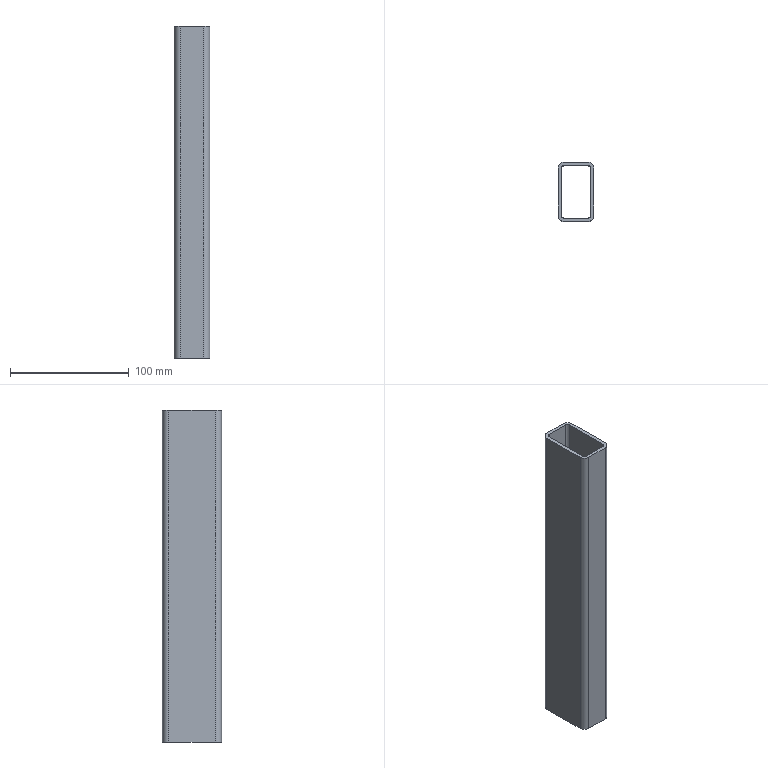Component | SolidWorks | Frame-1_SquareTube11-1 | 1 solid | 18 faces | box 30 x 50 x 280 mm | volume 104034 mm3 | plane 10 | cylinder 8 | commonest cylinder face diameters 5.2 x4 10.4 x4
STEP:
#1=COLOUR_RGB('',0.7922,0.8196,0.9333);
#2=FILL_AREA_STYLE_COLOUR('',#1);
#3=FILL_AREA_STYLE('',(#2));
#4=SURFACE_STYLE_FILL_AREA(#3);
#5=SURFACE_SIDE_STYLE('',(#4));
#6=SURFACE_STYLE_USAGE(.BOTH.,#5);
#7=PRESENTATION_STYLE_ASSIGNMENT((#6));
#8=CARTESIAN_POINT('',(-19.197,-11.622,-5.512));
#9=VERTEX_POINT('',#8);
#10=CARTESIAN_POINT('',(-19.197,-13.181,-5.512));
#11=VERTEX_POINT('',#10);
#12=CARTESIAN_POINT('',(-19.197,-11.622,-5.512));
#13=DIRECTION('',(0.,-1.,0.));
#14=VECTOR('',#13,39.37);
#15=LINE('',#12,#14);
#16=EDGE_CURVE('',#9,#11,#15,.T.);
#17=ORIENTED_EDGE('',*,*,#16,.T.);
#18=CARTESIAN_POINT('',(-19.197,-13.181,5.512));
#19=VERTEX_POINT('',#18);
#20=CARTESIAN_POINT('',(-19.197,-13.181,6.89));
#21=DIRECTION('',(0.,0.,1.));
#22=VECTOR('',#21,39.37);
#23=LINE('',#20,#22);
#24=EDGE_CURVE('',#11,#19,#23,.T.);
#25=ORIENTED_EDGE('',*,*,#24,.T.);
#26=CARTESIAN_POINT('',(-19.197,-11.622,5.512));
#27=VERTEX_POINT('',#26);
#28=CARTESIAN_POINT('',(-19.197,-11.622,5.512));
#29=DIRECTION('',(0.,1.,0.));
#30=VECTOR('',#29,39.37);
#31=LINE('',#28,#30);
#32=EDGE_CURVE('',#19,#27,#31,.T.);
#33=ORIENTED_EDGE('',*,*,#32,.T.);
#34=CARTESIAN_POINT('',(-19.197,-11.622,6.89));
#35=DIRECTION('',(-0.,0.,-1.));
#36=VECTOR('',#35,39.37);
#37=LINE('',#34,#36);
#38=EDGE_CURVE('',#27,#9,#37,.T.);
#39=ORIENTED_EDGE('',*,*,#38,.T.);
#40=EDGE_LOOP('',(#17,#25,#33,#39));
#41=FACE_OUTER_BOUND('',#40,.T.);
#42=CARTESIAN_POINT('',(-19.197,-11.622,6.89));
#43=DIRECTION('',(-1.,0.,0.));
#44=DIRECTION('',(0.,0.,1.));
#45=AXIS2_PLACEMENT_3D('',#42,#43,#44);
#46=PLANE('',#45);
#47=ADVANCED_FACE('',(#41),#46,.T.);
#48=ORIENTED_EDGE('',*,*,#24,.F.);
#49=CARTESIAN_POINT('',(-19.299,-13.283,-5.512));
#50=VERTEX_POINT('',#49);
#51=CARTESIAN_POINT('',(-19.299,-13.181,-5.512));
#52=DIRECTION('',(0.,0.,1.));
#53=DIRECTION('',(-1.,0.,0.));
#54=AXIS2_PLACEMENT_3D('',#51,#52,#53);
#55=CIRCLE('',#54,0.1024);
#56=EDGE_CURVE('',#50,#11,#55,.T.);
#57=ORIENTED_EDGE('',*,*,#56,.F.);
#58=CARTESIAN_POINT('',(-19.299,-13.283,5.512));
#59=VERTEX_POINT('',#58);
#60=CARTESIAN_POINT('',(-19.299,-13.283,6.89));
#61=DIRECTION('',(-0.,0.,-1.));
#62=VECTOR('',#61,39.37);
#63=LINE('',#60,#62);
#64=EDGE_CURVE('',#59,#50,#63,.T.);
#65=ORIENTED_EDGE('',*,*,#64,.F.);
#66=CARTESIAN_POINT('',(-19.299,-13.181,5.512));
#67=DIRECTION('',(-0.,0.,-1.));
#68=DIRECTION('',(-1.,0.,0.));
#69=AXIS2_PLACEMENT_3D('',#66,#67,#68);
#70=CIRCLE('',#69,0.1024);
#71=EDGE_CURVE('',#19,#59,#70,.T.);
#72=ORIENTED_EDGE('',*,*,#71,.F.);
#73=EDGE_LOOP('',(#48,#57,#65,#72));
#74=FACE_OUTER_BOUND('',#73,.T.);
#75=CARTESIAN_POINT('',(-19.299,-13.181,6.89));
#76=DIRECTION('',(-0.,0.,-1.));
#77=DIRECTION('',(-1.,0.,0.));
#78=AXIS2_PLACEMENT_3D('',#75,#76,#77);
#79=CYLINDRICAL_SURFACE('',#78,0.1024);
#80=ADVANCED_FACE('',(#74),#79,.F.);
#81=CARTESIAN_POINT('',(-19.299,-13.386,-5.512));
#82=VERTEX_POINT('',#81);
#83=CARTESIAN_POINT('',(-19.094,-13.181,-5.512));
#84=VERTEX_POINT('',#83);
#85=CARTESIAN_POINT('',(-19.299,-13.181,-5.512));
#86=DIRECTION('',(0.,0.,1.));
#87=DIRECTION('',(-1.,0.,0.));
#88=AXIS2_PLACEMENT_3D('',#85,#86,#87);
#89=CIRCLE('',#88,0.2047);
#90=EDGE_CURVE('',#82,#84,#89,.T.);
#91=ORIENTED_EDGE('',*,*,#90,.F.);
#92=CARTESIAN_POINT('',(-20.071,-13.386,-5.512));
#93=VERTEX_POINT('',#92);
#94=CARTESIAN_POINT('',(19.685,-13.386,-5.512));
#95=DIRECTION('',(1.,0.,0.));
#96=VECTOR('',#95,39.37);
#97=LINE('',#94,#96);
#98=EDGE_CURVE('',#93,#82,#97,.T.);
#99=ORIENTED_EDGE('',*,*,#98,.F.);
#100=CARTESIAN_POINT('',(-20.276,-13.181,-5.512));
#101=VERTEX_POINT('',#100);
#102=CARTESIAN_POINT('',(-20.071,-13.181,-5.512));
#103=DIRECTION('',(0.,0.,1.));
#104=DIRECTION('',(-1.,0.,0.));
#105=AXIS2_PLACEMENT_3D('',#102,#103,#104);
#106=CIRCLE('',#105,0.2047);
#107=EDGE_CURVE('',#101,#93,#106,.T.);
#108=ORIENTED_EDGE('',*,*,#107,.F.);
#109=CARTESIAN_POINT('',(-20.276,-11.622,-5.512));
#110=VERTEX_POINT('',#109);
#111=CARTESIAN_POINT('',(-20.276,-10.335,-5.512));
#112=DIRECTION('',(0.,-1.,0.));
#113=VECTOR('',#112,39.37);
#114=LINE('',#111,#113);
#115=EDGE_CURVE('',#110,#101,#114,.T.);
#116=ORIENTED_EDGE('',*,*,#115,.F.);
#117=CARTESIAN_POINT('',(-20.071,-11.417,-5.512));
#118=VERTEX_POINT('',#117);
#119=CARTESIAN_POINT('',(-20.071,-11.622,-5.512));
#120=DIRECTION('',(0.,0.,1.));
#121=DIRECTION('',(-1.,0.,0.));
#122=AXIS2_PLACEMENT_3D('',#119,#120,#121);
#123=CIRCLE('',#122,0.2047);
#124=EDGE_CURVE('',#118,#110,#123,.T.);
#125=ORIENTED_EDGE('',*,*,#124,.F.);
#126=CARTESIAN_POINT('',(-19.299,-11.417,-5.512));
#127=VERTEX_POINT('',#126);
#128=CARTESIAN_POINT('',(19.685,-11.417,-5.512));
#129=DIRECTION('',(-1.,0.,0.));
#130=VECTOR('',#129,39.37);
#131=LINE('',#128,#130);
#132=EDGE_CURVE('',#127,#118,#131,.T.);
#133=ORIENTED_EDGE('',*,*,#132,.F.);
#134=CARTESIAN_POINT('',(-19.094,-11.622,-5.512));
#135=VERTEX_POINT('',#134);
#136=CARTESIAN_POINT('',(-19.299,-11.622,-5.512));
#137=DIRECTION('',(0.,0.,1.));
#138=DIRECTION('',(-1.,0.,0.));
#139=AXIS2_PLACEMENT_3D('',#136,#137,#138);
#140=CIRCLE('',#139,0.2047);
#141=EDGE_CURVE('',#135,#127,#140,.T.);
#142=ORIENTED_EDGE('',*,*,#141,.F.);
#143=CARTESIAN_POINT('',(-19.094,-10.335,-5.512));
#144=DIRECTION('',(0.,1.,0.));
#145=VECTOR('',#144,39.37);
#146=LINE('',#143,#145);
#147=EDGE_CURVE('',#84,#135,#146,.T.);
#148=ORIENTED_EDGE('',*,*,#147,.F.);
#149=EDGE_LOOP('',(#91,#99,#108,#116,#125,#133,#142,#148));
#150=FACE_OUTER_BOUND('',#149,.T.);
#151=CARTESIAN_POINT('',(-20.173,-13.181,-5.512));
#152=VERTEX_POINT('',#151);
#153=CARTESIAN_POINT('',(-20.173,-11.622,-5.512));
#154=VERTEX_POINT('',#153);
#155=CARTESIAN_POINT('',(-20.173,-10.335,-5.512));
#156=DIRECTION('',(0.,1.,0.));
#157=VECTOR('',#156,39.37);
#158=LINE('',#155,#157);
#159=EDGE_CURVE('',#152,#154,#158,.T.);
#160=ORIENTED_EDGE('',*,*,#159,.F.);
#161=CARTESIAN_POINT('',(-20.071,-13.283,-5.512));
#162=VERTEX_POINT('',#161);
#163=CARTESIAN_POINT('',(-20.071,-13.181,-5.512));
#164=DIRECTION('',(-0.,0.,-1.));
#165=DIRECTION('',(-1.,0.,0.));
#166=AXIS2_PLACEMENT_3D('',#163,#164,#165);
#167=CIRCLE('',#166,0.1024);
#168=EDGE_CURVE('',#162,#152,#167,.T.);
#169=ORIENTED_EDGE('',*,*,#168,.F.);
#170=CARTESIAN_POINT('',(19.685,-13.283,-5.512));
#171=DIRECTION('',(-1.,0.,0.));
#172=VECTOR('',#171,39.37);
#173=LINE('',#170,#172);
#174=EDGE_CURVE('',#50,#162,#173,.T.);
#175=ORIENTED_EDGE('',*,*,#174,.F.);
#176=ORIENTED_EDGE('',*,*,#56,.T.);
#177=ORIENTED_EDGE('',*,*,#16,.F.);
#178=CARTESIAN_POINT('',(-19.299,-11.52,-5.512));
#179=VERTEX_POINT('',#178);
#180=CARTESIAN_POINT('',(-19.299,-11.622,-5.512));
#181=DIRECTION('',(-0.,0.,-1.));
#182=DIRECTION('',(-1.,0.,0.));
#183=AXIS2_PLACEMENT_3D('',#180,#181,#182);
#184=CIRCLE('',#183,0.1024);
#185=EDGE_CURVE('',#179,#9,#184,.T.);
#186=ORIENTED_EDGE('',*,*,#185,.F.);
#187=CARTESIAN_POINT('',(-20.071,-11.52,-5.512));
#188=VERTEX_POINT('',#187);
#189=CARTESIAN_POINT('',(19.685,-11.52,-5.512));
#190=DIRECTION('',(1.,0.,0.));
#191=VECTOR('',#190,39.37);
#192=LINE('',#189,#191);
#193=EDGE_CURVE('',#188,#179,#192,.T.);
#194=ORIENTED_EDGE('',*,*,#193,.F.);
#195=CARTESIAN_POINT('',(-20.071,-11.622,-5.512));
#196=DIRECTION('',(-0.,0.,-1.));
#197=DIRECTION('',(-1.,0.,0.));
#198=AXIS2_PLACEMENT_3D('',#195,#196,#197);
#199=CIRCLE('',#198,0.1024);
#200=EDGE_CURVE('',#154,#188,#199,.T.);
#201=ORIENTED_EDGE('',*,*,#200,.F.);
#202=EDGE_LOOP('',(#160,#169,#175,#176,#177,#186,#194,#201));
#203=FACE_BOUND('',#202,.T.);
#204=CARTESIAN_POINT('',(19.685,-10.335,-5.512));
#205=DIRECTION('',(0.,0.,1.));
#206=DIRECTION('',(1.,0.,0.));
#207=AXIS2_PLACEMENT_3D('',#204,#205,#206);
#208=PLANE('',#207);
#209=ADVANCED_FACE('',(#150,#203),#208,.F.);
#210=CARTESIAN_POINT('',(-19.299,-11.52,5.512));
#211=VERTEX_POINT('',#210);
#212=CARTESIAN_POINT('',(-19.299,-11.52,6.89));
#213=DIRECTION('',(0.,0.,1.));
#214=VECTOR('',#213,39.37);
#215=LINE('',#212,#214);
#216=EDGE_CURVE('',#179,#211,#215,.T.);
#217=ORIENTED_EDGE('',*,*,#216,.F.);
#218=ORIENTED_EDGE('',*,*,#185,.T.);
#219=ORIENTED_EDGE('',*,*,#38,.F.);
#220=CARTESIAN_POINT('',(-19.299,-11.622,5.512));
#221=DIRECTION('',(-0.,0.,-1.));
#222=DIRECTION('',(-1.,0.,0.));
#223=AXIS2_PLACEMENT_3D('',#220,#221,#222);
#224=CIRCLE('',#223,0.1024);
#225=EDGE_CURVE('',#211,#27,#224,.T.);
#226=ORIENTED_EDGE('',*,*,#225,.F.);
#227=EDGE_LOOP('',(#217,#218,#219,#226));
#228=FACE_OUTER_BOUND('',#227,.T.);
#229=CARTESIAN_POINT('',(-19.299,-11.622,6.89));
#230=DIRECTION('',(-0.,0.,-1.));
#231=DIRECTION('',(-1.,0.,0.));
#232=AXIS2_PLACEMENT_3D('',#229,#230,#231);
#233=CYLINDRICAL_SURFACE('',#232,0.1024);
#234=ADVANCED_FACE('',(#228),#233,.F.);
#235=CARTESIAN_POINT('',(-20.071,-11.417,5.512));
#236=VERTEX_POINT('',#235);
#237=CARTESIAN_POINT('',(-19.299,-11.417,5.512));
#238=VERTEX_POINT('',#237);
#239=CARTESIAN_POINT('',(19.685,-11.417,5.512));
#240=DIRECTION('',(1.,0.,0.));
#241=VECTOR('',#240,39.37);
#242=LINE('',#239,#241);
#243=EDGE_CURVE('',#236,#238,#242,.T.);
#244=ORIENTED_EDGE('',*,*,#243,.F.);
#245=CARTESIAN_POINT('',(-20.276,-11.622,5.512));
#246=VERTEX_POINT('',#245);
#247=CARTESIAN_POINT('',(-20.071,-11.622,5.512));
#248=DIRECTION('',(-0.,0.,-1.));
#249=DIRECTION('',(-1.,0.,0.));
#250=AXIS2_PLACEMENT_3D('',#247,#248,#249);
#251=CIRCLE('',#250,0.2047);
#252=EDGE_CURVE('',#246,#236,#251,.T.);
#253=ORIENTED_EDGE('',*,*,#252,.F.);
#254=CARTESIAN_POINT('',(-20.276,-13.181,5.512));
#255=VERTEX_POINT('',#254);
#256=CARTESIAN_POINT('',(-20.276,-10.335,5.512));
#257=DIRECTION('',(0.,1.,0.));
#258=VECTOR('',#257,39.37);
#259=LINE('',#256,#258);
#260=EDGE_CURVE('',#255,#246,#259,.T.);
#261=ORIENTED_EDGE('',*,*,#260,.F.);
#262=CARTESIAN_POINT('',(-20.071,-13.386,5.512));
#263=VERTEX_POINT('',#262);
#264=CARTESIAN_POINT('',(-20.071,-13.181,5.512));
#265=DIRECTION('',(-0.,0.,-1.));
#266=DIRECTION('',(-1.,0.,0.));
#267=AXIS2_PLACEMENT_3D('',#264,#265,#266);
#268=CIRCLE('',#267,0.2047);
#269=EDGE_CURVE('',#263,#255,#268,.T.);
#270=ORIENTED_EDGE('',*,*,#269,.F.);
#271=CARTESIAN_POINT('',(-19.299,-13.386,5.512));
#272=VERTEX_POINT('',#271);
#273=CARTESIAN_POINT('',(19.685,-13.386,5.512));
#274=DIRECTION('',(-1.,0.,0.));
#275=VECTOR('',#274,39.37);
#276=LINE('',#273,#275);
#277=EDGE_CURVE('',#272,#263,#276,.T.);
#278=ORIENTED_EDGE('',*,*,#277,.F.);
#279=CARTESIAN_POINT('',(-19.094,-13.181,5.512));
#280=VERTEX_POINT('',#279);
#281=CARTESIAN_POINT('',(-19.299,-13.181,5.512));
#282=DIRECTION('',(-0.,0.,-1.));
#283=DIRECTION('',(-1.,0.,0.));
#284=AXIS2_PLACEMENT_3D('',#281,#282,#283);
#285=CIRCLE('',#284,0.2047);
#286=EDGE_CURVE('',#280,#272,#285,.T.);
#287=ORIENTED_EDGE('',*,*,#286,.F.);
#288=CARTESIAN_POINT('',(-19.094,-11.622,5.512));
#289=VERTEX_POINT('',#288);
#290=CARTESIAN_POINT('',(-19.094,-10.335,5.512));
#291=DIRECTION('',(0.,-1.,0.));
#292=VECTOR('',#291,39.37);
#293=LINE('',#290,#292);
#294=EDGE_CURVE('',#289,#280,#293,.T.);
#295=ORIENTED_EDGE('',*,*,#294,.F.);
#296=CARTESIAN_POINT('',(-19.299,-11.622,5.512));
#297=DIRECTION('',(-0.,0.,-1.));
#298=DIRECTION('',(-1.,0.,0.));
#299=AXIS2_PLACEMENT_3D('',#296,#297,#298);
#300=CIRCLE('',#299,0.2047);
#301=EDGE_CURVE('',#238,#289,#300,.T.);
#302=ORIENTED_EDGE('',*,*,#301,.F.);
#303=EDGE_LOOP('',(#244,#253,#261,#270,#278,#287,#295,#302));
#304=FACE_OUTER_BOUND('',#303,.T.);
#305=CARTESIAN_POINT('',(-20.071,-11.52,5.512));
#306=VERTEX_POINT('',#305);
#307=CARTESIAN_POINT('',(-20.173,-11.622,5.512));
#308=VERTEX_POINT('',#307);
#309=CARTESIAN_POINT('',(-20.071,-11.622,5.512));
#310=DIRECTION('',(0.,0.,1.));
#311=DIRECTION('',(-1.,0.,0.));
#312=AXIS2_PLACEMENT_3D('',#309,#310,#311);
#313=CIRCLE('',#312,0.1024);
#314=EDGE_CURVE('',#306,#308,#313,.T.);
#315=ORIENTED_EDGE('',*,*,#314,.F.);
#316=CARTESIAN_POINT('',(19.685,-11.52,5.512));
#317=DIRECTION('',(-1.,0.,0.));
#318=VECTOR('',#317,39.37);
#319=LINE('',#316,#318);
#320=EDGE_CURVE('',#211,#306,#319,.T.);
#321=ORIENTED_EDGE('',*,*,#320,.F.);
#322=ORIENTED_EDGE('',*,*,#225,.T.);
#323=ORIENTED_EDGE('',*,*,#32,.F.);
#324=ORIENTED_EDGE('',*,*,#71,.T.);
#325=CARTESIAN_POINT('',(-20.071,-13.283,5.512));
#326=VERTEX_POINT('',#325);
#327=CARTESIAN_POINT('',(19.685,-13.283,5.512));
#328=DIRECTION('',(1.,0.,0.));
#329=VECTOR('',#328,39.37);
#330=LINE('',#327,#329);
#331=EDGE_CURVE('',#326,#59,#330,.T.);
#332=ORIENTED_EDGE('',*,*,#331,.F.);
#333=CARTESIAN_POINT('',(-20.173,-13.181,5.512));
#334=VERTEX_POINT('',#333);
#335=CARTESIAN_POINT('',(-20.071,-13.181,5.512));
#336=DIRECTION('',(0.,0.,1.));
#337=DIRECTION('',(-1.,0.,0.));
#338=AXIS2_PLACEMENT_3D('',#335,#336,#337);
#339=CIRCLE('',#338,0.1024);
#340=EDGE_CURVE('',#334,#326,#339,.T.);
#341=ORIENTED_EDGE('',*,*,#340,.F.);
#342=CARTESIAN_POINT('',(-20.173,-10.335,5.512));
#343=DIRECTION('',(0.,-1.,0.));
#344=VECTOR('',#343,39.37);
#345=LINE('',#342,#344);
#346=EDGE_CURVE('',#308,#334,#345,.T.);
#347=ORIENTED_EDGE('',*,*,#346,.F.);
#348=EDGE_LOOP('',(#315,#321,#322,#323,#324,#332,#341,#347));
#349=FACE_BOUND('',#348,.T.);
#350=CARTESIAN_POINT('',(19.685,-10.335,5.512));
#351=DIRECTION('',(0.,0.,-1.));
#352=DIRECTION('',(-1.,0.,0.));
#353=AXIS2_PLACEMENT_3D('',#350,#351,#352);
#354=PLANE('',#353);
#355=ADVANCED_FACE('',(#304,#349),#354,.F.);
#356=ORIENTED_EDGE('',*,*,#174,.T.);
#357=CARTESIAN_POINT('',(-20.071,-13.283,6.89));
#358=DIRECTION('',(0.,0.,1.));
#359=VECTOR('',#358,39.37);
#360=LINE('',#357,#359);
#361=EDGE_CURVE('',#162,#326,#360,.T.);
#362=ORIENTED_EDGE('',*,*,#361,.T.);
#363=ORIENTED_EDGE('',*,*,#331,.T.);
#364=ORIENTED_EDGE('',*,*,#64,.T.);
#365=EDGE_LOOP('',(#356,#362,#363,#364));
#366=FACE_OUTER_BOUND('',#365,.T.);
#367=CARTESIAN_POINT('',(-20.071,-13.283,6.89));
#368=DIRECTION('',(0.,1.,0.));
#369=DIRECTION('',(0.,0.,1.));
#370=AXIS2_PLACEMENT_3D('',#367,#368,#369);
#371=PLANE('',#370);
#372=ADVANCED_FACE('',(#366),#371,.T.);
#373=ORIENTED_EDGE('',*,*,#294,.T.);
#374=CARTESIAN_POINT('',(-19.094,-13.181,6.89));
#375=DIRECTION('',(0.,0.,1.));
#376=VECTOR('',#375,39.37);
#377=LINE('',#374,#376);
#378=EDGE_CURVE('',#84,#280,#377,.T.);
#379=ORIENTED_EDGE('',*,*,#378,.F.);
#380=ORIENTED_EDGE('',*,*,#147,.T.);
#381=CARTESIAN_POINT('',(-19.094,-11.622,6.89));
#382=DIRECTION('',(-0.,0.,-1.));
#383=VECTOR('',#382,39.37);
#384=LINE('',#381,#383);
#385=EDGE_CURVE('',#289,#135,#384,.T.);
#386=ORIENTED_EDGE('',*,*,#385,.F.);
#387=EDGE_LOOP('',(#373,#379,#380,#386));
#388=FACE_OUTER_BOUND('',#387,.T.);
#389=CARTESIAN_POINT('',(-19.094,-11.622,6.89));
#390=DIRECTION('',(-1.,0.,0.));
#391=DIRECTION('',(0.,0.,1.));
#392=AXIS2_PLACEMENT_3D('',#389,#390,#391);
#393=PLANE('',#392);
#394=ADVANCED_FACE('',(#388),#393,.F.);
#395=CARTESIAN_POINT('',(-19.299,-13.386,6.89));
#396=DIRECTION('',(-0.,0.,-1.));
#397=VECTOR('',#396,39.37);
#398=LINE('',#395,#397);
#399=EDGE_CURVE('',#272,#82,#398,.T.);
#400=ORIENTED_EDGE('',*,*,#399,.T.);
#401=ORIENTED_EDGE('',*,*,#90,.T.);
#402=ORIENTED_EDGE('',*,*,#378,.T.);
#403=ORIENTED_EDGE('',*,*,#286,.T.);
#404=EDGE_LOOP('',(#400,#401,#402,#403));
#405=FACE_OUTER_BOUND('',#404,.T.);
#406=CARTESIAN_POINT('',(-19.299,-13.181,6.89));
#407=DIRECTION('',(-0.,0.,-1.));
#408=DIRECTION('',(-1.,0.,0.));
#409=AXIS2_PLACEMENT_3D('',#406,#407,#408);
#410=CYLINDRICAL_SURFACE('',#409,0.2047);
#411=ADVANCED_FACE('',(#405),#410,.T.);
#412=ORIENTED_EDGE('',*,*,#277,.T.);
#413=CARTESIAN_POINT('',(-20.071,-13.386,6.89));
#414=DIRECTION('',(0.,0.,1.));
#415=VECTOR('',#414,39.37);
#416=LINE('',#413,#415);
#417=EDGE_CURVE('',#93,#263,#416,.T.);
#418=ORIENTED_EDGE('',*,*,#417,.F.);
#419=ORIENTED_EDGE('',*,*,#98,.T.);
#420=ORIENTED_EDGE('',*,*,#399,.F.);
#421=EDGE_LOOP('',(#412,#418,#419,#420));
#422=FACE_OUTER_BOUND('',#421,.T.);
#423=CARTESIAN_POINT('',(-20.071,-13.386,6.89));
#424=DIRECTION('',(0.,1.,0.));
#425=DIRECTION('',(0.,0.,1.));
#426=AXIS2_PLACEMENT_3D('',#423,#424,#425);
#427=PLANE('',#426);
#428=ADVANCED_FACE('',(#422),#427,.F.);
#429=CARTESIAN_POINT('',(-20.276,-13.181,6.89));
#430=DIRECTION('',(-0.,0.,-1.));
#431=VECTOR('',#430,39.37);
#432=LINE('',#429,#431);
#433=EDGE_CURVE('',#255,#101,#432,.T.);
#434=ORIENTED_EDGE('',*,*,#433,.T.);
#435=ORIENTED_EDGE('',*,*,#107,.T.);
#436=ORIENTED_EDGE('',*,*,#417,.T.);
#437=ORIENTED_EDGE('',*,*,#269,.T.);
#438=EDGE_LOOP('',(#434,#435,#436,#437));
#439=FACE_OUTER_BOUND('',#438,.T.);
#440=CARTESIAN_POINT('',(-20.071,-13.181,6.89));
#441=DIRECTION('',(-0.,0.,-1.));
#442=DIRECTION('',(-1.,0.,0.));
#443=AXIS2_PLACEMENT_3D('',#440,#441,#442);
#444=CYLINDRICAL_SURFACE('',#443,0.2047);
#445=ADVANCED_FACE('',(#439),#444,.T.);
#446=ORIENTED_EDGE('',*,*,#260,.T.);
#447=CARTESIAN_POINT('',(-20.276,-11.622,6.89));
#448=DIRECTION('',(0.,0.,1.));
#449=VECTOR('',#448,39.37);
#450=LINE('',#447,#449);
#451=EDGE_CURVE('',#110,#246,#450,.T.);
#452=ORIENTED_EDGE('',*,*,#451,.F.);
#453=ORIENTED_EDGE('',*,*,#115,.T.);
#454=ORIENTED_EDGE('',*,*,#433,.F.);
#455=EDGE_LOOP('',(#446,#452,#453,#454));
#456=FACE_OUTER_BOUND('',#455,.T.);
#457=CARTESIAN_POINT('',(-20.276,-13.181,6.89));
#458=DIRECTION('',(1.,0.,-0.));
#459=DIRECTION('',(-0.,0.,-1.));
#460=AXIS2_PLACEMENT_3D('',#457,#458,#459);
#461=PLANE('',#460);
#462=ADVANCED_FACE('',(#456),#461,.F.);
#463=CARTESIAN_POINT('',(-20.071,-11.417,6.89));
#464=DIRECTION('',(-0.,0.,-1.));
#465=VECTOR('',#464,39.37);
#466=LINE('',#463,#465);
#467=EDGE_CURVE('',#236,#118,#466,.T.);
#468=ORIENTED_EDGE('',*,*,#467,.T.);
#469=ORIENTED_EDGE('',*,*,#124,.T.);
#470=ORIENTED_EDGE('',*,*,#451,.T.);
#471=ORIENTED_EDGE('',*,*,#252,.T.);
#472=EDGE_LOOP('',(#468,#469,#470,#471));
#473=FACE_OUTER_BOUND('',#472,.T.);
#474=CARTESIAN_POINT('',(-20.071,-11.622,6.89));
#475=DIRECTION('',(-0.,0.,-1.));
#476=DIRECTION('',(-1.,0.,0.));
#477=AXIS2_PLACEMENT_3D('',#474,#475,#476);
#478=CYLINDRICAL_SURFACE('',#477,0.2047);
#479=ADVANCED_FACE('',(#473),#478,.T.);
#480=ORIENTED_EDGE('',*,*,#243,.T.);
#481=CARTESIAN_POINT('',(-19.299,-11.417,6.89));
#482=DIRECTION('',(0.,0.,1.));
#483=VECTOR('',#482,39.37);
#484=LINE('',#481,#483);
#485=EDGE_CURVE('',#127,#238,#484,.T.);
#486=ORIENTED_EDGE('',*,*,#485,.F.);
#487=ORIENTED_EDGE('',*,*,#132,.T.);
#488=ORIENTED_EDGE('',*,*,#467,.F.);
#489=EDGE_LOOP('',(#480,#486,#487,#488));
#490=FACE_OUTER_BOUND('',#489,.T.);
#491=CARTESIAN_POINT('',(-19.299,-11.417,6.89));
#492=DIRECTION('',(0.,-1.,0.));
#493=DIRECTION('',(0.,0.,-1.));
#494=AXIS2_PLACEMENT_3D('',#491,#492,#493);
#495=PLANE('',#494);
#496=ADVANCED_FACE('',(#490),#495,.F.);
#497=ORIENTED_EDGE('',*,*,#385,.T.);
#498=ORIENTED_EDGE('',*,*,#141,.T.);
#499=ORIENTED_EDGE('',*,*,#485,.T.);
#500=ORIENTED_EDGE('',*,*,#301,.T.);
#501=EDGE_LOOP('',(#497,#498,#499,#500));
#502=FACE_OUTER_BOUND('',#501,.T.);
#503=CARTESIAN_POINT('',(-19.299,-11.622,6.89));
#504=DIRECTION('',(-0.,0.,-1.));
#505=DIRECTION('',(-1.,0.,0.));
#506=AXIS2_PLACEMENT_3D('',#503,#504,#505);
#507=CYLINDRICAL_SURFACE('',#506,0.2047);
#508=ADVANCED_FACE('',(#502),#507,.T.);
#509=CARTESIAN_POINT('',(-20.173,-11.622,6.89));
#510=DIRECTION('',(0.,0.,1.));
#511=VECTOR('',#510,39.37);
#512=LINE('',#509,#511);
#513=EDGE_CURVE('',#154,#308,#512,.T.);
#514=ORIENTED_EDGE('',*,*,#513,.F.);
#515=ORIENTED_EDGE('',*,*,#200,.T.);
#516=CARTESIAN_POINT('',(-20.071,-11.52,6.89));
#517=DIRECTION('',(-0.,0.,-1.));
#518=VECTOR('',#517,39.37);
#519=LINE('',#516,#518);
#520=EDGE_CURVE('',#306,#188,#519,.T.);
#521=ORIENTED_EDGE('',*,*,#520,.F.);
#522=ORIENTED_EDGE('',*,*,#314,.T.);
#523=EDGE_LOOP('',(#514,#515,#521,#522));
#524=FACE_OUTER_BOUND('',#523,.T.);
#525=CARTESIAN_POINT('',(-20.071,-11.622,6.89));
#526=DIRECTION('',(-0.,0.,-1.));
#527=DIRECTION('',(-1.,0.,0.));
#528=AXIS2_PLACEMENT_3D('',#525,#526,#527);
#529=CYLINDRICAL_SURFACE('',#528,0.1024);
#530=ADVANCED_FACE('',(#524),#529,.F.);
#531=ORIENTED_EDGE('',*,*,#159,.T.);
#532=ORIENTED_EDGE('',*,*,#513,.T.);
#533=ORIENTED_EDGE('',*,*,#346,.T.);
#534=CARTESIAN_POINT('',(-20.173,-13.181,6.89));
#535=DIRECTION('',(-0.,0.,-1.));
#536=VECTOR('',#535,39.37);
#537=LINE('',#534,#536);
#538=EDGE_CURVE('',#334,#152,#537,.T.);
#539=ORIENTED_EDGE('',*,*,#538,.T.);
#540=EDGE_LOOP('',(#531,#532,#533,#539));
#541=FACE_OUTER_BOUND('',#540,.T.);
#542=CARTESIAN_POINT('',(-20.173,-13.181,6.89));
#543=DIRECTION('',(1.,0.,-0.));
#544=DIRECTION('',(-0.,0.,-1.));
#545=AXIS2_PLACEMENT_3D('',#542,#543,#544);
#546=PLANE('',#545);
#547=ADVANCED_FACE('',(#541),#546,.T.);
#548=ORIENTED_EDGE('',*,*,#361,.F.);
#549=ORIENTED_EDGE('',*,*,#168,.T.);
#550=ORIENTED_EDGE('',*,*,#538,.F.);
#551=ORIENTED_EDGE('',*,*,#340,.T.);
#552=EDGE_LOOP('',(#548,#549,#550,#551));
#553=FACE_OUTER_BOUND('',#552,.T.);
#554=CARTESIAN_POINT('',(-20.071,-13.181,6.89));
#555=DIRECTION('',(-0.,0.,-1.));
#556=DIRECTION('',(-1.,0.,0.));
#557=AXIS2_PLACEMENT_3D('',#554,#555,#556);
#558=CYLINDRICAL_SURFACE('',#557,0.1024);
#559=ADVANCED_FACE('',(#553),#558,.F.);
#560=ORIENTED_EDGE('',*,*,#193,.T.);
#561=ORIENTED_EDGE('',*,*,#216,.T.);
#562=ORIENTED_EDGE('',*,*,#320,.T.);
#563=ORIENTED_EDGE('',*,*,#520,.T.);
#564=EDGE_LOOP('',(#560,#561,#562,#563));
#565=FACE_OUTER_BOUND('',#564,.T.);
#566=CARTESIAN_POINT('',(-19.299,-11.52,6.89));
#567=DIRECTION('',(0.,-1.,0.));
#568=DIRECTION('',(0.,0.,-1.));
#569=AXIS2_PLACEMENT_3D('',#566,#567,#568);
#570=PLANE('',#569);
#571=ADVANCED_FACE('',(#565),#570,.T.);
#572=CLOSED_SHELL('',(#47,#80,#209,#234,#355,#372,#394,#411,#428,#445,#462,#479,#496,#508,#530,#547,#559,#571));
#573=MANIFOLD_SOLID_BREP('',#572);
#574=STYLED_ITEM('',(#7),#573);
#575=PRESENTATION_LAYER_ASSIGNMENT('','',(#574));
#576=CARTESIAN_POINT('',(0.,0.,0.));
#577=DIRECTION('',(0.,0.,1.));
#578=DIRECTION('',(1.,0.,0.));
#579=AXIS2_PLACEMENT_3D('',#576,#577,#578);
#580=(LENGTH_UNIT()NAMED_UNIT(*)SI_UNIT($,.METRE.));
#581=LENGTH_MEASURE_WITH_UNIT(LENGTH_MEASURE(0.0254),#580);
#582=DIMENSIONAL_EXPONENTS(1.,0.,0.,0.,0.,0.,0.);
#583=(CONVERSION_BASED_UNIT('',#581)LENGTH_UNIT()NAMED_UNIT(#582));
#584=UNCERTAINTY_MEASURE_WITH_UNIT(LENGTH_MEASURE(0.00001),#583,'','');
#585=(NAMED_UNIT(*)PLANE_ANGLE_UNIT()SI_UNIT($,.RADIAN.));
#586=(NAMED_UNIT(*)SI_UNIT($,.STERADIAN.)SOLID_ANGLE_UNIT());
#587=(GEOMETRIC_REPRESENTATION_CONTEXT(3)GLOBAL_UNCERTAINTY_ASSIGNED_CONTEXT((#584))GLOBAL_UNIT_ASSIGNED_CONTEXT((#583,#585,#586))REPRESENTATION_CONTEXT('',''));
#588=ADVANCED_BREP_SHAPE_REPRESENTATION('',(#573,#579),#587);
#589=(LENGTH_UNIT()NAMED_UNIT(*)SI_UNIT($,.METRE.));
#590=LENGTH_MEASURE_WITH_UNIT(LENGTH_MEASURE(0.0254),#589);
#591=DIMENSIONAL_EXPONENTS(1.,0.,0.,0.,0.,0.,0.);
#592=(CONVERSION_BASED_UNIT('',#590)LENGTH_UNIT()NAMED_UNIT(#591));
#593=UNCERTAINTY_MEASURE_WITH_UNIT(LENGTH_MEASURE(0.00001),#592,'','');
#594=(NAMED_UNIT(*)PLANE_ANGLE_UNIT()SI_UNIT($,.RADIAN.));
#595=(NAMED_UNIT(*)SI_UNIT($,.STERADIAN.)SOLID_ANGLE_UNIT());
#596=(GEOMETRIC_REPRESENTATION_CONTEXT(3)GLOBAL_UNCERTAINTY_ASSIGNED_CONTEXT((#593))GLOBAL_UNIT_ASSIGNED_CONTEXT((#592,#594,#595))REPRESENTATION_CONTEXT('',''));
#597=MECHANICAL_DESIGN_GEOMETRIC_PRESENTATION_REPRESENTATION('',(#574),#596);